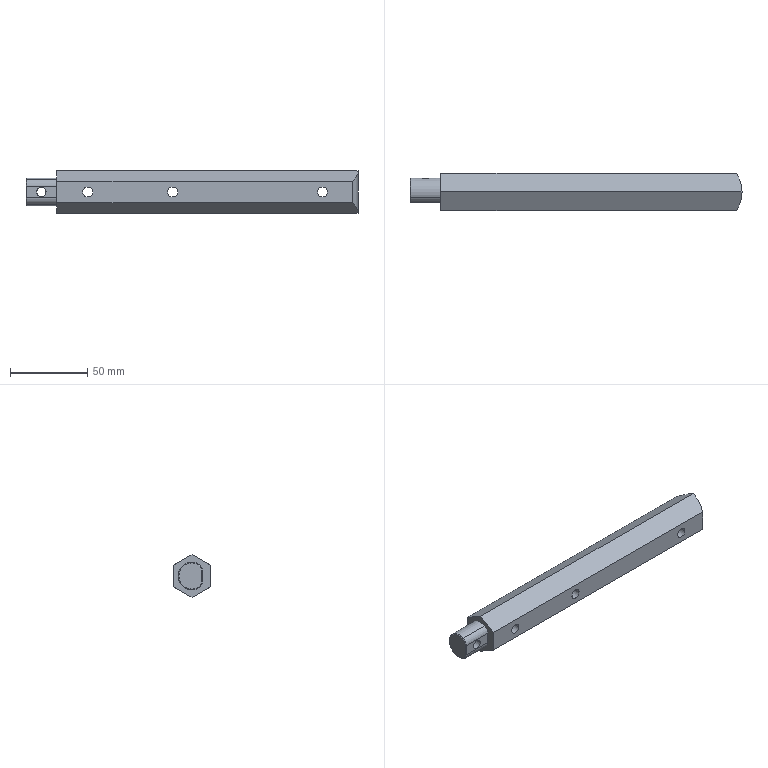Component | SolidWorks | LowerReceiver-1 | 1 solid | 36 faces | box 215 x 24 x 27.71 mm | volume 95513 mm3 | cylinder 19 | plane 13 | cone 4 | commonest cylinder face diameters 12 x6 6.5 x6 6 x2 18 x2 10 x2 44 x1
build123d program:
from build123d import *

# Parameters (mm, degrees)
BOSS_EXTRUDE1_DEPTH                                 = 195
BOSS_EXTRUDE2_DEPTH                                 = 20
CYLINDRICAL_COUNTERSUNK_HOLE_FOR_M6_HEX_D           = 6.5
CYLINDRICAL_COUNTERSUNK_HOLE_FOR_M6_HEX_CBORE_D     = 12
CYLINDRICAL_COUNTERSUNK_HOLE_FOR_M6_HEX_CBORE_DEPTH = 15
CYLINDRICAL_COUNTERSUNK_HOLE_FOR_M6_2_D             = 6.5
CYLINDRICAL_COUNTERSUNK_HOLE_FOR_M6_2_CBORE_D       = 12
CYLINDRICAL_COUNTERSUNK_HOLE_FOR_M6_2_CBORE_DEPTH   = 12
SKETCH17_R                                          = 3
CUT_EXTRUDE2_DEPTH                                  = 20
CUT_EXTRUDE3_DEPTH                                  = 216.78
CUT_EXTRUDE3_DEPTH_BACK                             = 216.78
CHAMFER1_SIZE                                       = 0.5


with BuildPart() as part:
    # Sketch1 → Boss-Extrude1 (new body)
    with BuildSketch(Plane.XY):
        Polygon((12, -6.928), (12, 6.928), (0, 13.856), (-12, 6.928), (-12, -6.928), (0, -13.856), align=None)
    extrude(amount=BOSS_EXTRUDE1_DEPTH)

    # Sketch2 → Boss-Extrude2 (add)
    with BuildSketch(Plane.XY.offset(195)):
        with BuildLine():
            Line((6.7, 3.621), (6.7, -3.621))
            ThreePointArc((6.7, -3.621), (5.92, -6.302), (3.825, -8.147))
            ThreePointArc((3.825, -8.147), (-9, 0), (3.825, 8.147))
            ThreePointArc((3.825, 8.147), (5.92, 6.302), (6.7, 3.621))
        make_face()
    extrude(amount=BOSS_EXTRUDE2_DEPTH)

    # Cylindrical Countersunk Hole for M6 Hex (through all)
    with Locations(Plane.ZY.offset(12)):
        with Locations((23, 0)):
            CounterBoreHole(CYLINDRICAL_COUNTERSUNK_HOLE_FOR_M6_HEX_D / 2, CYLINDRICAL_COUNTERSUNK_HOLE_FOR_M6_HEX_CBORE_D / 2, CYLINDRICAL_COUNTERSUNK_HOLE_FOR_M6_HEX_CBORE_DEPTH)

    # Cylindrical Countersunk Hole for M6  2 (through all)
    with Locations(Plane.ZY.offset(12)):
        with Locations((175, 0), (120, 0)):
            CounterBoreHole(CYLINDRICAL_COUNTERSUNK_HOLE_FOR_M6_2_D / 2, CYLINDRICAL_COUNTERSUNK_HOLE_FOR_M6_2_CBORE_D / 2, CYLINDRICAL_COUNTERSUNK_HOLE_FOR_M6_2_CBORE_DEPTH)

    # Sketch17 → Cut-Extrude2 (cut)
    with BuildSketch(Plane(origin=(-9, 0, 0), x_dir=(0, 0, -1), z_dir=(1, 0, 0))):
        with Locations(Location((-205, 0, 0), (0, 0, 180))):
            Circle(SKETCH17_R)
    extrude(amount=CUT_EXTRUDE2_DEPTH, mode=Mode.SUBTRACT)

    # Sketch18 → Cut-Extrude3 (cut, two sides: drawn at the far end of the back side and taken through both)
    with BuildSketch(Plane(origin=(0, 0, 0), x_dir=(1, 0, 0), z_dir=(0, 1, 0)).offset(-CUT_EXTRUDE3_DEPTH_BACK)):
        with BuildLine():
            Line((-12, 0), (-12, -3.561))
            ThreePointArc((-12, -3.561), (-6.259, -0.909), (0, 0))
            Line((0, 0), (-12, 0))
        make_face()
        with BuildLine():
            Line((12, 0), (0, 0))
            ThreePointArc((0, 0), (6.259, -0.909), (12, -3.561))
            Line((12, -3.561), (12, 0))
        make_face()
    extrude(amount=CUT_EXTRUDE3_DEPTH + CUT_EXTRUDE3_DEPTH_BACK, mode=Mode.SUBTRACT)

    # Chamfer1
    chamfer1_edges = [part.edges().sort_by_distance(p)[0] for p in [
        (5.92, -6.302, 215),
        (6.7, 0, 215),
        (5.92, 6.302, 215),
        (-9, 0, 215),
    ]]
    chamfer(chamfer1_edges, length=CHAMFER1_SIZE)


solid = part.part

# Placed as in the assembly
solid = solid.moved(Location((224.182, 34.483, 1009), (90, -90, 0)))